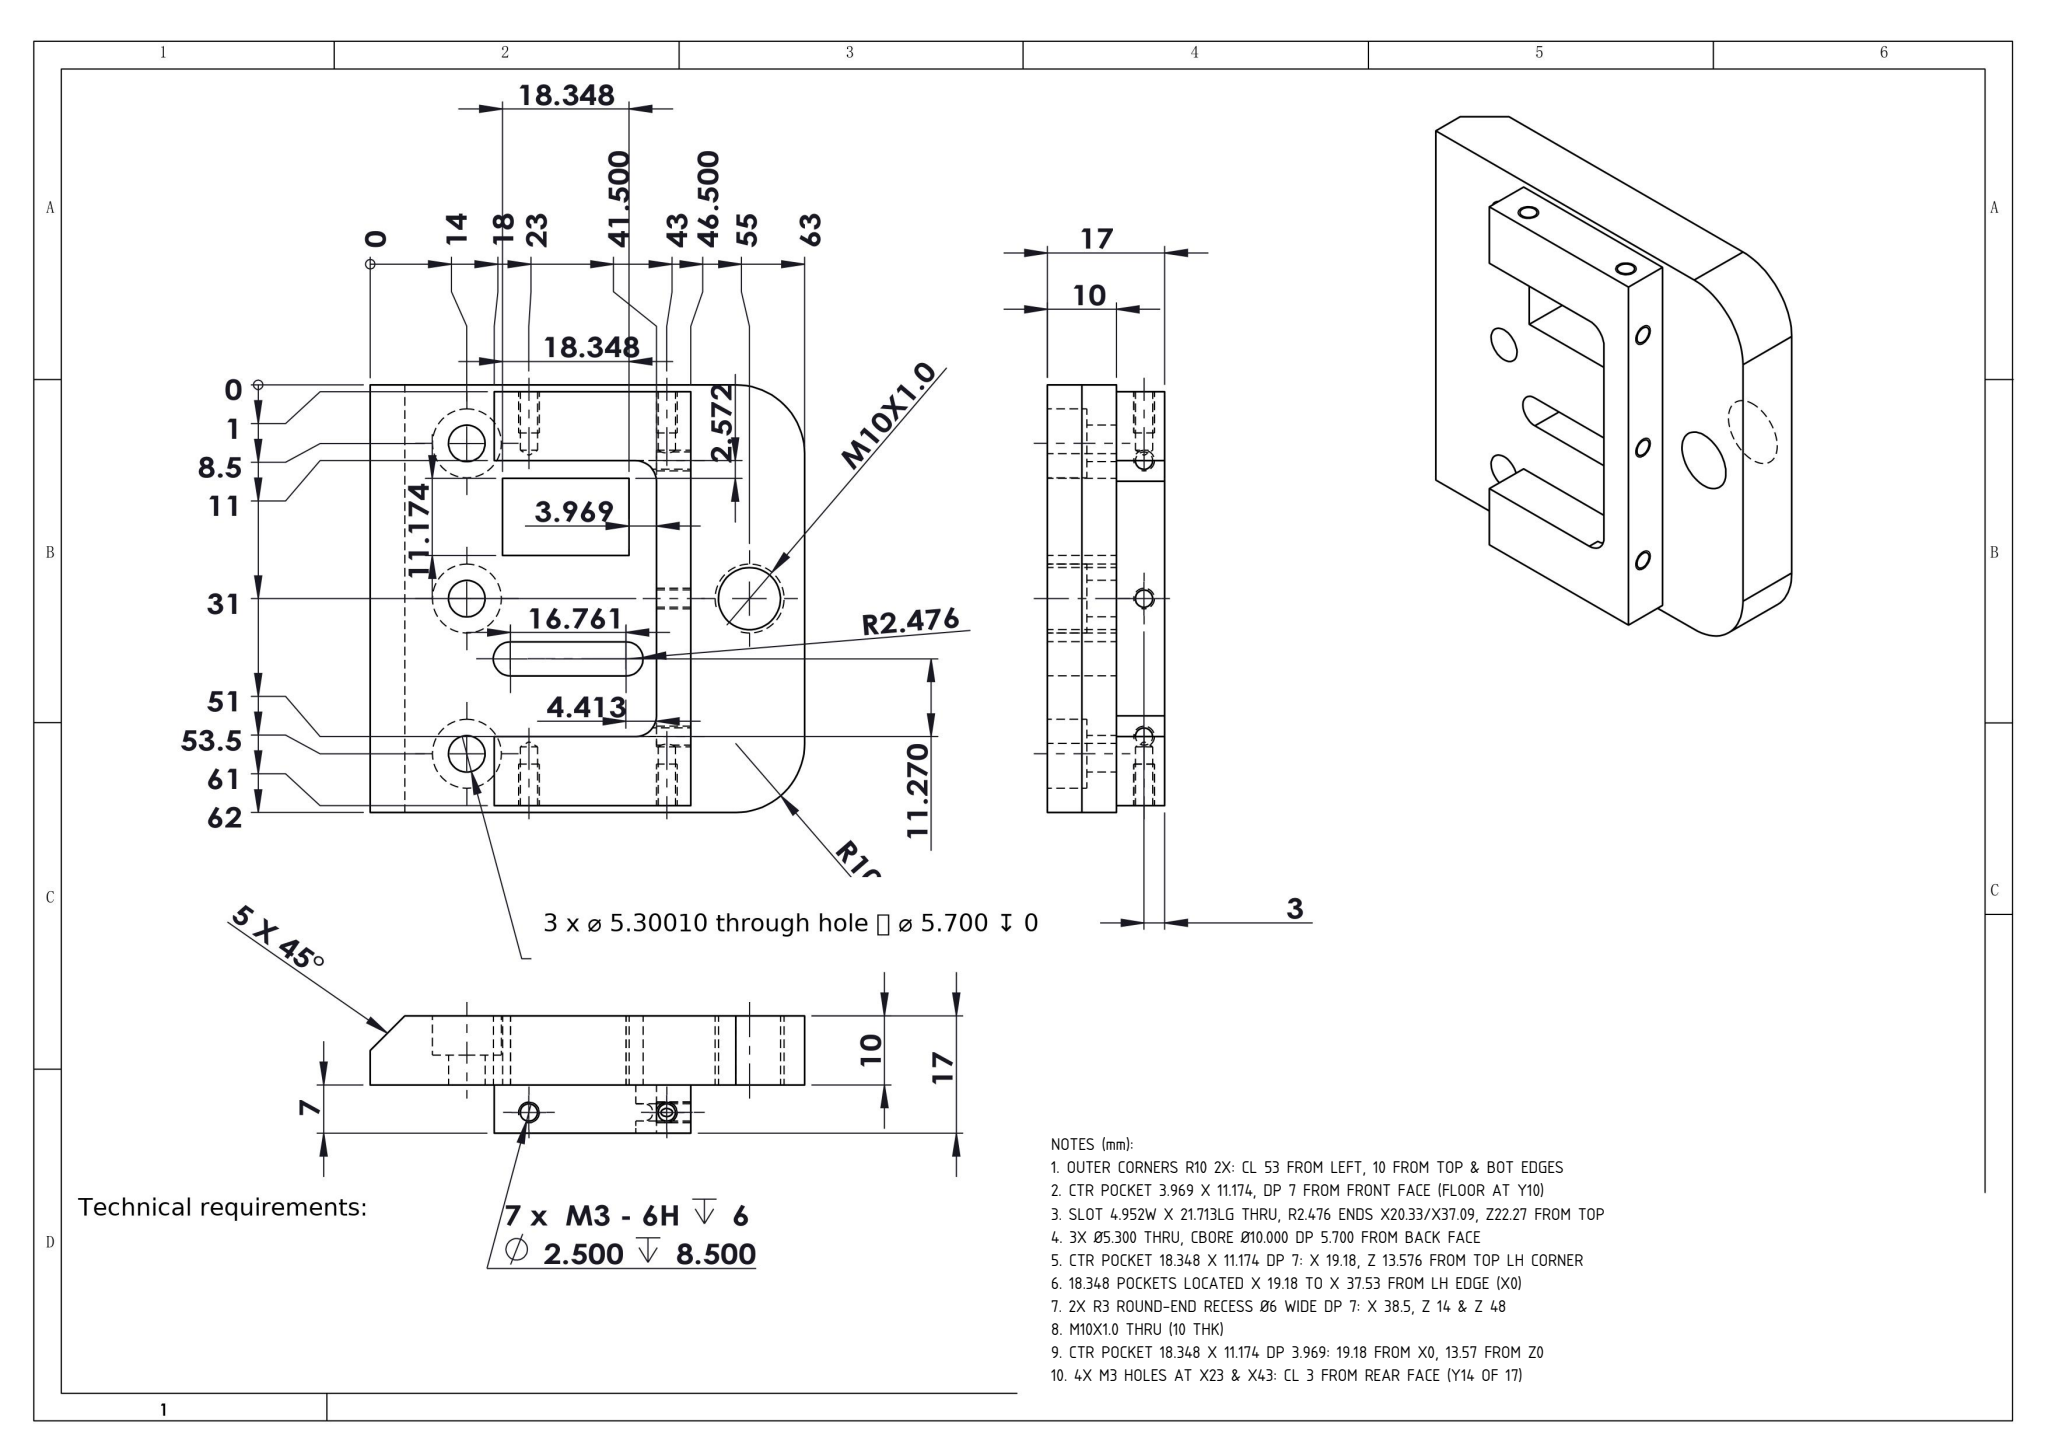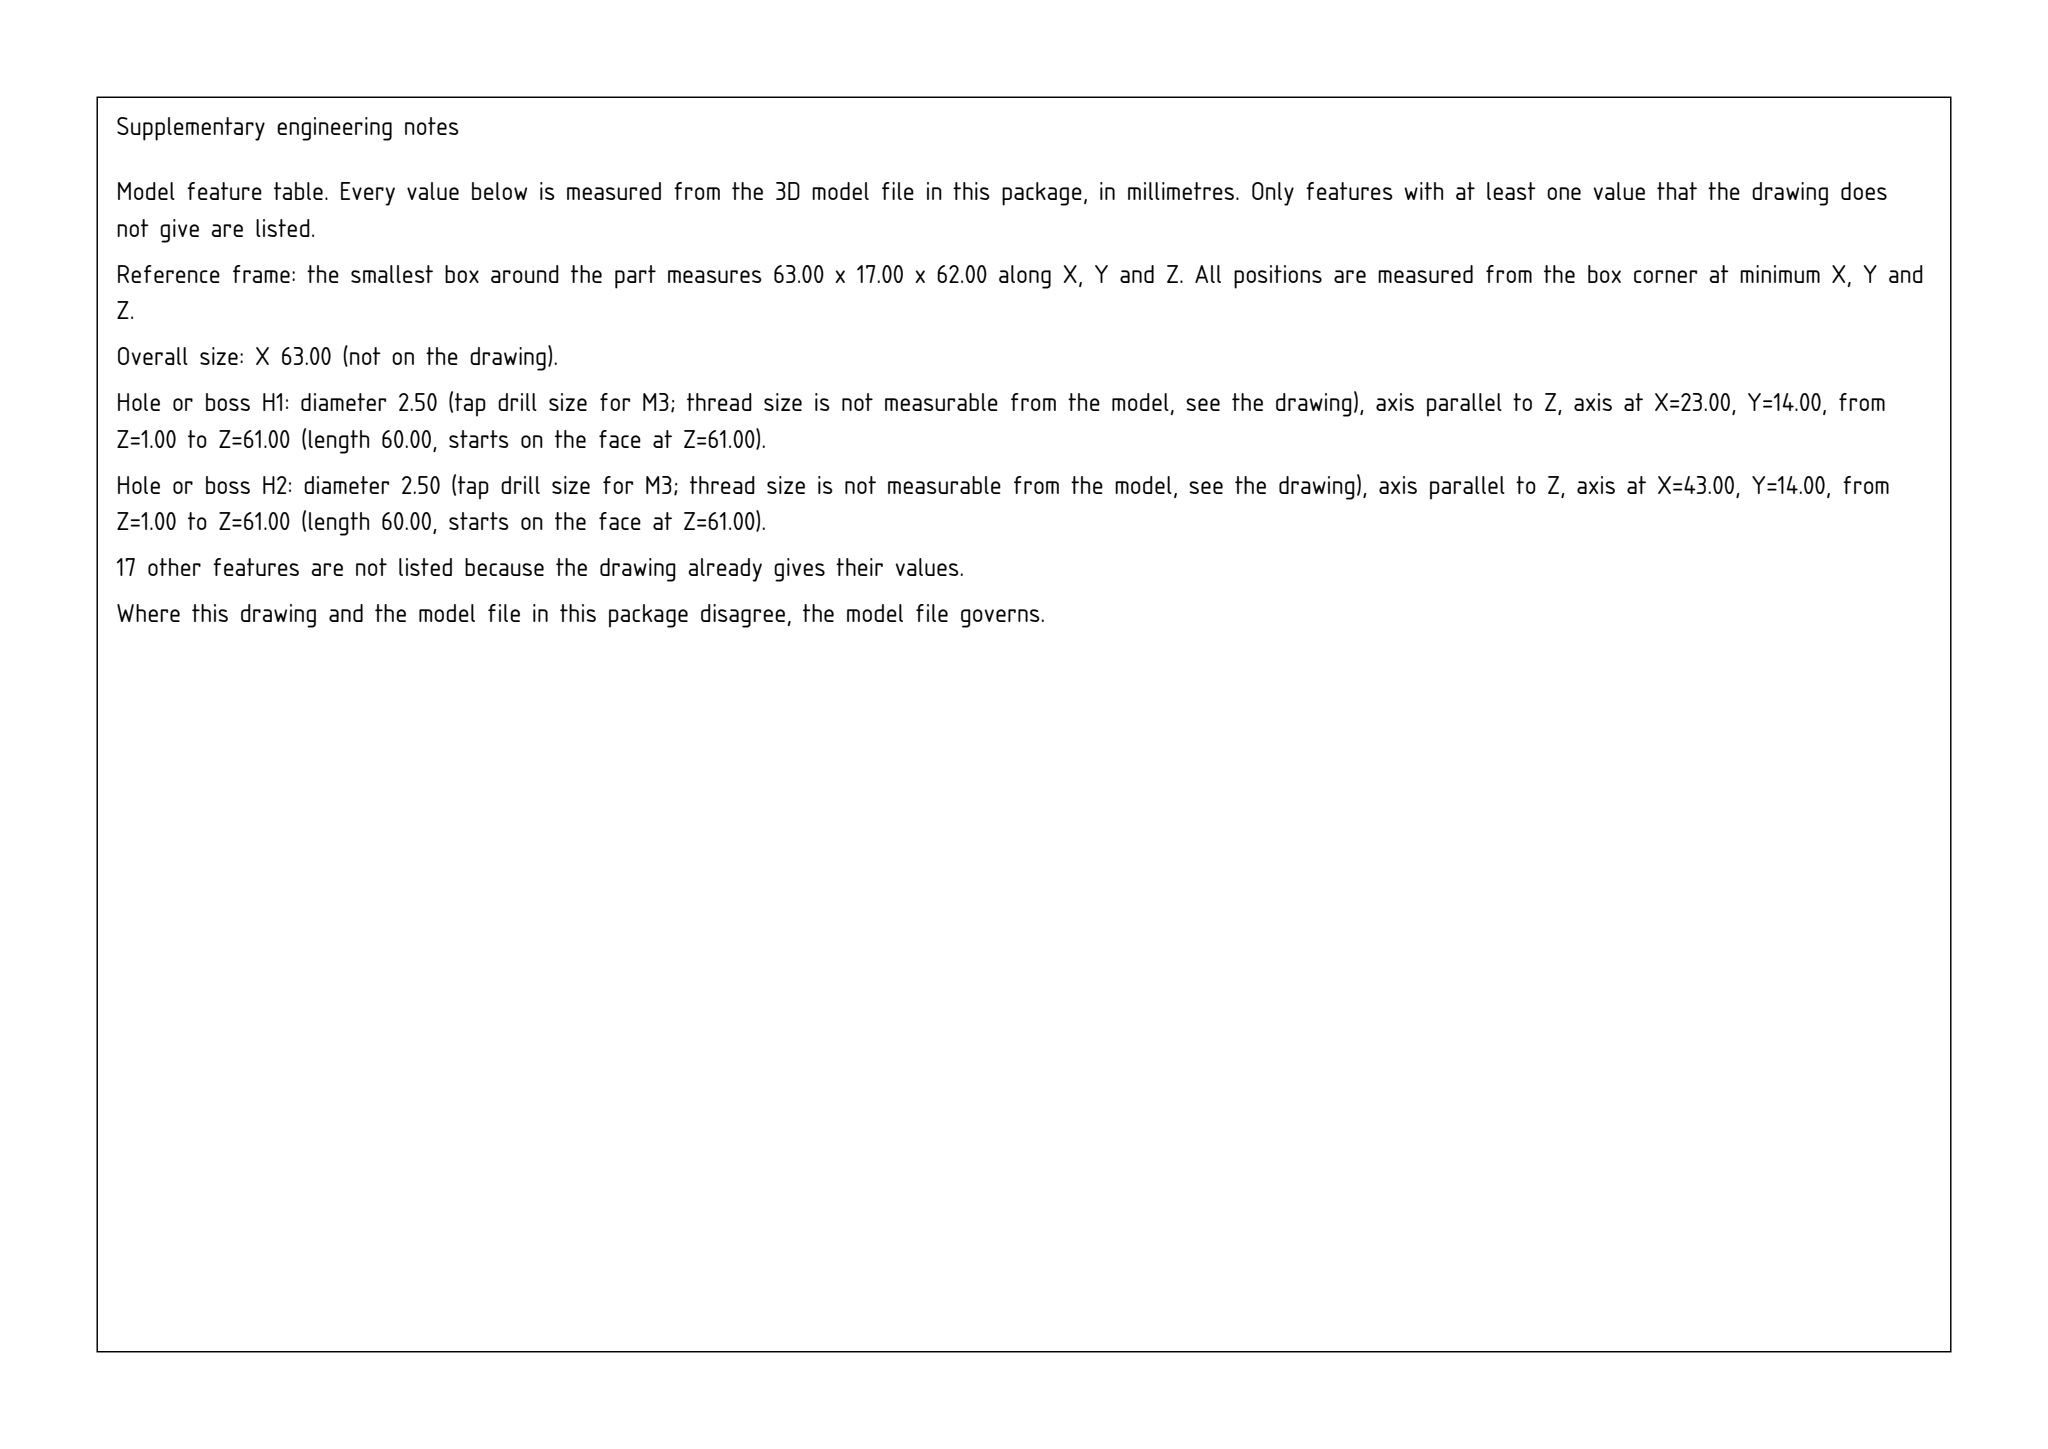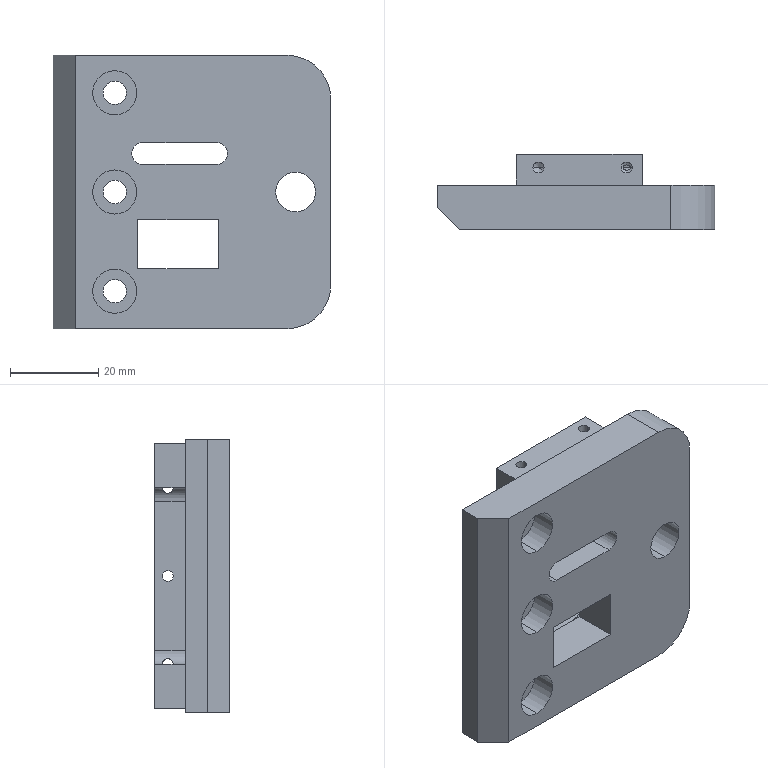Part | SolidWorks | mm | 1 solid | 69 faces | box 63 x 17 x 62 mm | volume 37684 mm3 | cylinder 34 | plane 27 | cone 8 | commonest cylinder face diameters 2.5 x14 10 x6 5.3 x6 9 x2 20 x2 6 x2 4.952 x2
Drawing notes:
OUTER CORNERS R10 2X: CL 53 FROM LEFT, 10 FROM TOP & BOT EDGES | from the solid: Ø20.0 axis-Y cyls at (x53,z10) and (x53,z52), len 10 = 2 corner rounds R10 thru 10 thk plate
CTR POCKET 3.969 X 11.174, DP 7 FROM FRONT FACE (FLOOR AT Y10) | from the solid: Only internal y-plane besides cbores is y=10.0; front face y=17.0, so floor 7.0 below front
SLOT 4.952W X 21.713LG THRU, R2.476 ENDS X20.33/X37.09, Z22.27 FROM TOP | from the solid: Two Ø4.952 axis-Y cyls at (20.33,39.73) & (37.09,39.73), len 10 thru; ctr dist 16.76; 62-39.73=22.27
3X Ø5.300 THRU, CBORE Ø10.000 DP 5.700 FROM BACK FACE | from the solid: Ø5.3 axis-Y len 4.3 at x14, z8.5/31/53.5 coaxial with Ø10.0 axis-Y len 5.7; y-plane 5.7 = cbore floor
CTR POCKET 18.348 X 11.174 DP 7: X 19.18, Z 13.576 FROM TOP LH CORNER | from the solid: x planes 19.18 & 37.53 (18.348), z planes 13.57 & 24.75 (11.174), y 17->10 = 7 deep
18.348 POCKETS LOCATED X 19.18 TO X 37.53 FROM LH EDGE (X0) | from the solid: axis_planes x=19.18 and x=37.53; 37.53-19.18=18.348; bbox x origin 0
2X R3 ROUND-END RECESS Ø6 WIDE DP 7: X 38.5, Z 14 & Z 48 | from the solid: cylinders [6.0,'y',[38.5,null,14.0],7.0] and [6.0,'y',[38.5,null,48.0],7.0]
M10X1.0 THRU (10 THK) | from the solid: cyl [9.0,'y',[55.0,null,31.0],10.0]; y planes 0 and 10 = full local thickness
CTR POCKET 18.348 X 11.174 DP 3.969: 19.18 FROM X0, 13.57 FROM Z0 | from the solid: x-planes 19.18 & 37.53 (18.35 wide), z-planes 13.57 & 24.75 (11.18 tall), pocket depth 3.969 from front face
4X M3 HOLES AT X23 & X43: CL 3 FROM REAR FACE (Y14 OF 17) | from the solid: Ø2.5 z-axis cyls at (23,14) and (43,14), L8.5; bbox Y=17 so 17-14=3